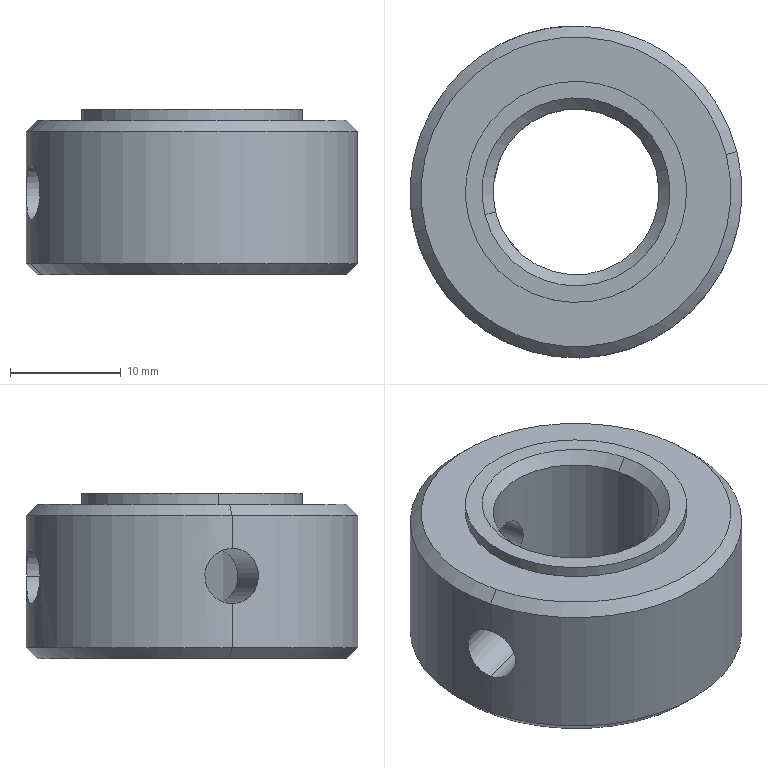Component | SolidWorks | KSD171005A-01-01-28-1 | 1 solid | 21 faces | box 30 x 30 x 15 mm | volume 7121 mm3 | cylinder 10 | cone 8 | plane 3 | commonest cylinder face diameters 5 x4 15 x2 20 x2 30 x2
build123d program:
from build123d import *

# Parameters (mm, degrees)
CHAMFER1_SIZE = 1
CHAMFER2_SIZE = 1
SKETCH2_W     = 2.5
SKETCH2_H     = 15
SKETCH4_W     = 2.5
SKETCH4_H     = 15


with BuildPart() as part:
    # Sketch1 → Revolve1 (revolve)
    with BuildSketch(Plane.XY, mode=Mode.PRIVATE) as revolve1_sk:
        Polygon((-7.5, 7.5), (7.5, 7.5), (7.5, 10), (6.5, 10), (6.5, 15), (-7.5, 15), align=None)
    revolve(revolve1_sk.sketch.rotate(Axis((0, 0, 0), (-1, 0, 0)), 90), axis=Axis((0, 0, 0), (-1, 0, 0)))

    # Chamfer1
    chamfer1_edges = [part.edges().sort_by_distance(p)[0] for p in [
        (6.5, 0, 15),
        (-7.5, 0, 15),
    ]]
    chamfer(chamfer1_edges, length=CHAMFER1_SIZE)

    # Chamfer2
    chamfer2_edges = [part.edges().sort_by_distance(p)[0] for p in [
        (-7.5, 0, 7.5),
        (7.5, 0, 7.5),
    ]]
    chamfer(chamfer2_edges, length=CHAMFER2_SIZE)

    # Sketch2 → M6 Tapped Hole1 (revolve, cut)
    with BuildSketch(Plane(origin=(0, 0, 0), x_dir=(0, 0, -1), z_dir=(1, 0, 0))):
        with Locations((1.25, 7.5)):
            Rectangle(SKETCH2_W, SKETCH2_H)
    revolve(axis=Axis((0, -6.35, 0), (0, 1, 0)), mode=Mode.SUBTRACT)

    # Sketch4 → M6 Tapped Hole2 (revolve, cut)
    with BuildSketch(Plane.YZ):
        with Locations((1.25, 7.5)):
            Rectangle(SKETCH4_W, SKETCH4_H)
    revolve(axis=Axis((0, 0, -6.35), (0, 0, 1)), mode=Mode.SUBTRACT)


solid = part.part

# Placed as in the assembly
solid = solid.moved(Location((-7.111, 15.73, 340.5), (90, -75.982, 90)))
STEP:
#1=COLOUR_RGB('',0.7922,0.8196,0.9333);
#2=FILL_AREA_STYLE_COLOUR('',#1);
#3=FILL_AREA_STYLE('',(#2));
#4=SURFACE_STYLE_FILL_AREA(#3);
#5=SURFACE_SIDE_STYLE('',(#4));
#6=SURFACE_STYLE_USAGE(.BOTH.,#5);
#7=PRESENTATION_STYLE_ASSIGNMENT((#6));
#8=CARTESIAN_POINT('',(-0.8529,0.4762,13.307));
#9=VERTEX_POINT('',#8);
#10=CARTESIAN_POINT('',(-0.8529,0.4762,13.504));
#11=VERTEX_POINT('',#10);
#12=CARTESIAN_POINT('',(-0.8529,0.4762,13.307));
#13=CARTESIAN_POINT('',(-0.8514,0.4699,13.307));
#14=CARTESIAN_POINT('',(-0.8497,0.4637,13.308));
#15=CARTESIAN_POINT('',(-0.8463,0.4516,13.31));
#16=CARTESIAN_POINT('',(-0.8444,0.4456,13.312));
#17=CARTESIAN_POINT('',(-0.8408,0.4342,13.317));
#18=CARTESIAN_POINT('',(-0.839,0.4288,13.32));
#19=CARTESIAN_POINT('',(-0.8354,0.4187,13.327));
#20=CARTESIAN_POINT('',(-0.8337,0.4139,13.331));
#21=CARTESIAN_POINT('',(-0.8288,0.4011,13.345));
#22=CARTESIAN_POINT('',(-0.826,0.3943,13.356));
#23=CARTESIAN_POINT('',(-0.8231,0.3874,13.374));
#24=CARTESIAN_POINT('',(-0.8224,0.3857,13.38));
#25=CARTESIAN_POINT('',(-0.8213,0.3833,13.393));
#26=CARTESIAN_POINT('',(-0.8211,0.3827,13.399));
#27=CARTESIAN_POINT('',(-0.8211,0.3827,13.412));
#28=CARTESIAN_POINT('',(-0.8213,0.3833,13.418));
#29=CARTESIAN_POINT('',(-0.8224,0.3857,13.431));
#30=CARTESIAN_POINT('',(-0.8231,0.3874,13.437));
#31=CARTESIAN_POINT('',(-0.825,0.392,13.449));
#32=CARTESIAN_POINT('',(-0.8262,0.3949,13.455));
#33=CARTESIAN_POINT('',(-0.8289,0.4015,13.466));
#34=CARTESIAN_POINT('',(-0.8304,0.4054,13.471));
#35=CARTESIAN_POINT('',(-0.8337,0.414,13.48));
#36=CARTESIAN_POINT('',(-0.8354,0.4187,13.484));
#37=CARTESIAN_POINT('',(-0.839,0.4288,13.491));
#38=CARTESIAN_POINT('',(-0.8408,0.4343,13.494));
#39=CARTESIAN_POINT('',(-0.8444,0.4456,13.499));
#40=CARTESIAN_POINT('',(-0.8462,0.4515,13.501));
#41=CARTESIAN_POINT('',(-0.8497,0.4637,13.503));
#42=CARTESIAN_POINT('',(-0.8514,0.47,13.504));
#43=CARTESIAN_POINT('',(-0.8529,0.4762,13.504));
#44=B_SPLINE_CURVE_WITH_KNOTS('',3,(#12,#13,#14,#15,#16,#17,#18,#19,#20,#21,#22,#23,#24,#25,#26,#27,#28,#29,#30,#31,#32,#33,#34,#35,#36,#37,#38,#39,#40,#41,#42,#43),.UNSPECIFIED.,.F.,.F.,(4,2,2,2,2,2,2,2,2,2,2,2,2,2,2,4),(0.,0.0004894,0.0009787,0.001468,0.001957,0.002936,0.003426,0.003915,0.004404,0.004894,0.005383,0.005872,0.006362,0.006851,0.00734,0.00783),.UNSPECIFIED.);
#45=EDGE_CURVE('',#9,#11,#44,.T.);
#46=ORIENTED_EDGE('',*,*,#45,.T.);
#47=CARTESIAN_POINT('',(-0.5665,0.5477,13.504));
#48=VERTEX_POINT('',#47);
#49=CARTESIAN_POINT('',(-0.28,0.6193,13.504));
#50=DIRECTION('',(0.9702,0.2423,0.));
#51=VECTOR('',#50,39.37);
#52=LINE('',#49,#51);
#53=EDGE_CURVE('',#11,#48,#52,.T.);
#54=ORIENTED_EDGE('',*,*,#53,.T.);
#55=CARTESIAN_POINT('',(-0.5665,0.5477,13.307));
#56=VERTEX_POINT('',#55);
#57=CARTESIAN_POINT('',(-0.5665,0.5477,13.504));
#58=CARTESIAN_POINT('',(-0.5649,0.5415,13.504));
#59=CARTESIAN_POINT('',(-0.5631,0.5352,13.503));
#60=CARTESIAN_POINT('',(-0.5592,0.523,13.501));
#61=CARTESIAN_POINT('',(-0.5571,0.5172,13.499));
#62=CARTESIAN_POINT('',(-0.5528,0.5061,13.494));
#63=CARTESIAN_POINT('',(-0.5505,0.5007,13.491));
#64=CARTESIAN_POINT('',(-0.5459,0.4909,13.484));
#65=CARTESIAN_POINT('',(-0.5437,0.4864,13.48));
#66=CARTESIAN_POINT('',(-0.5372,0.4739,13.466));
#67=CARTESIAN_POINT('',(-0.5333,0.4675,13.455));
#68=CARTESIAN_POINT('',(-0.5292,0.4608,13.437));
#69=CARTESIAN_POINT('',(-0.5281,0.4592,13.431));
#70=CARTESIAN_POINT('',(-0.5266,0.4569,13.419));
#71=CARTESIAN_POINT('',(-0.5262,0.4563,13.412));
#72=CARTESIAN_POINT('',(-0.5262,0.4563,13.399));
#73=CARTESIAN_POINT('',(-0.5266,0.4569,13.393));
#74=CARTESIAN_POINT('',(-0.5281,0.4592,13.38));
#75=CARTESIAN_POINT('',(-0.5292,0.4609,13.374));
#76=CARTESIAN_POINT('',(-0.5333,0.4675,13.356));
#77=CARTESIAN_POINT('',(-0.5372,0.474,13.345));
#78=CARTESIAN_POINT('',(-0.5437,0.4863,13.331));
#79=CARTESIAN_POINT('',(-0.546,0.4909,13.327));
#80=CARTESIAN_POINT('',(-0.5505,0.5008,13.32));
#81=CARTESIAN_POINT('',(-0.5527,0.506,13.317));
#82=CARTESIAN_POINT('',(-0.5571,0.5172,13.312));
#83=CARTESIAN_POINT('',(-0.5592,0.5231,13.31));
#84=CARTESIAN_POINT('',(-0.5631,0.5352,13.308));
#85=CARTESIAN_POINT('',(-0.5649,0.5414,13.307));
#86=CARTESIAN_POINT('',(-0.5665,0.5477,13.307));
#87=B_SPLINE_CURVE_WITH_KNOTS('',3,(#57,#58,#59,#60,#61,#62,#63,#64,#65,#66,#67,#68,#69,#70,#71,#72,#73,#74,#75,#76,#77,#78,#79,#80,#81,#82,#83,#84,#85,#86),.UNSPECIFIED.,.F.,.F.,(4,2,2,2,2,2,2,2,2,2,2,2,2,2,4),(0.007873,0.008365,0.008857,0.009349,0.009841,0.01082,0.01132,0.01181,0.0123,0.01279,0.01378,0.01427,0.01476,0.01525,0.01574),.UNSPECIFIED.);
#88=EDGE_CURVE('',#48,#56,#87,.T.);
#89=ORIENTED_EDGE('',*,*,#88,.T.);
#90=CARTESIAN_POINT('',(-0.28,0.6193,13.307));
#91=DIRECTION('',(0.9702,0.2423,0.));
#92=VECTOR('',#91,39.37);
#93=LINE('',#90,#92);
#94=EDGE_CURVE('',#9,#56,#93,.T.);
#95=ORIENTED_EDGE('',*,*,#94,.F.);
#96=EDGE_LOOP('',(#46,#54,#89,#95));
#97=FACE_OUTER_BOUND('',#96,.T.);
#98=CARTESIAN_POINT('',(-0.28,0.6193,13.406));
#99=DIRECTION('',(0.9702,0.2423,0.));
#100=DIRECTION('',(0.,0.,-1.));
#101=AXIS2_PLACEMENT_3D('',#98,#99,#100);
#102=CYLINDRICAL_SURFACE('',#101,0.09843);
#103=ADVANCED_FACE('',(#97),#102,.F.);
#104=CARTESIAN_POINT('',(-0.3255,1.208,13.406));
#105=VERTEX_POINT('',#104);
#106=CARTESIAN_POINT('',(-0.5165,1.16,13.406));
#107=VERTEX_POINT('',#106);
#108=CARTESIAN_POINT('',(-0.3255,1.208,13.406));
#109=CARTESIAN_POINT('',(-0.3255,1.208,13.399));
#110=CARTESIAN_POINT('',(-0.3262,1.208,13.393));
#111=CARTESIAN_POINT('',(-0.3287,1.208,13.38));
#112=CARTESIAN_POINT('',(-0.3306,1.208,13.374));
#113=CARTESIAN_POINT('',(-0.3356,1.207,13.362));
#114=CARTESIAN_POINT('',(-0.3387,1.207,13.356));
#115=CARTESIAN_POINT('',(-0.3458,1.206,13.345));
#116=CARTESIAN_POINT('',(-0.35,1.206,13.34));
#117=CARTESIAN_POINT('',(-0.3636,1.204,13.327));
#118=CARTESIAN_POINT('',(-0.3745,1.202,13.32));
#119=CARTESIAN_POINT('',(-0.392,1.199,13.312));
#120=CARTESIAN_POINT('',(-0.3981,1.198,13.31));
#121=CARTESIAN_POINT('',(-0.4105,1.195,13.308));
#122=CARTESIAN_POINT('',(-0.4168,1.194,13.307));
#123=CARTESIAN_POINT('',(-0.4292,1.191,13.307));
#124=CARTESIAN_POINT('',(-0.4356,1.189,13.308));
#125=CARTESIAN_POINT('',(-0.4477,1.186,13.31));
#126=CARTESIAN_POINT('',(-0.4536,1.184,13.312));
#127=CARTESIAN_POINT('',(-0.465,1.18,13.317));
#128=CARTESIAN_POINT('',(-0.4705,1.178,13.32));
#129=CARTESIAN_POINT('',(-0.4805,1.175,13.327));
#130=CARTESIAN_POINT('',(-0.4853,1.173,13.331));
#131=CARTESIAN_POINT('',(-0.4939,1.17,13.34));
#132=CARTESIAN_POINT('',(-0.4977,1.168,13.345));
#133=CARTESIAN_POINT('',(-0.5044,1.166,13.356));
#134=CARTESIAN_POINT('',(-0.5072,1.164,13.362));
#135=CARTESIAN_POINT('',(-0.5118,1.162,13.374));
#136=CARTESIAN_POINT('',(-0.5136,1.162,13.38));
#137=CARTESIAN_POINT('',(-0.5159,1.161,13.393));
#138=CARTESIAN_POINT('',(-0.5165,1.16,13.399));
#139=CARTESIAN_POINT('',(-0.5165,1.16,13.406));
#140=B_SPLINE_CURVE_WITH_KNOTS('',3,(#108,#109,#110,#111,#112,#113,#114,#115,#116,#117,#118,#119,#120,#121,#122,#123,#124,#125,#126,#127,#128,#129,#130,#131,#132,#133,#134,#135,#136,#137,#138,#139),.UNSPECIFIED.,.F.,.F.,(4,2,2,2,2,2,2,2,2,2,2,2,2,2,2,4),(0.,0.0004894,0.0009787,0.001468,0.001957,0.002936,0.003426,0.003915,0.004404,0.004894,0.005383,0.005872,0.006362,0.006851,0.00734,0.00783),.UNSPECIFIED.);
#141=EDGE_CURVE('',#105,#107,#140,.T.);
#142=ORIENTED_EDGE('',*,*,#141,.T.);
#143=CARTESIAN_POINT('',(-0.4429,0.8655,13.406));
#144=VERTEX_POINT('',#143);
#145=CARTESIAN_POINT('',(-0.3755,0.5954,13.406));
#146=DIRECTION('',(0.2423,-0.9702,0.));
#147=VECTOR('',#146,39.37);
#148=LINE('',#145,#147);
#149=EDGE_CURVE('',#107,#144,#148,.T.);
#150=ORIENTED_EDGE('',*,*,#149,.T.);
#151=CARTESIAN_POINT('',(-0.2519,0.9132,13.406));
#152=VERTEX_POINT('',#151);
#153=CARTESIAN_POINT('',(-0.4429,0.8655,13.406));
#154=CARTESIAN_POINT('',(-0.4429,0.8655,13.399));
#155=CARTESIAN_POINT('',(-0.4423,0.8659,13.393));
#156=CARTESIAN_POINT('',(-0.4401,0.8674,13.38));
#157=CARTESIAN_POINT('',(-0.4384,0.8685,13.374));
#158=CARTESIAN_POINT('',(-0.434,0.8712,13.362));
#159=CARTESIAN_POINT('',(-0.4312,0.8729,13.356));
#160=CARTESIAN_POINT('',(-0.4248,0.8766,13.345));
#161=CARTESIAN_POINT('',(-0.4212,0.8787,13.34));
#162=CARTESIAN_POINT('',(-0.4087,0.8852,13.327));
#163=CARTESIAN_POINT('',(-0.3988,0.8898,13.32));
#164=CARTESIAN_POINT('',(-0.382,0.8964,13.312));
#165=CARTESIAN_POINT('',(-0.3762,0.8985,13.31));
#166=CARTESIAN_POINT('',(-0.3641,0.9024,13.308));
#167=CARTESIAN_POINT('',(-0.3578,0.9042,13.307));
#168=CARTESIAN_POINT('',(-0.3452,0.9073,13.307));
#169=CARTESIAN_POINT('',(-0.3389,0.9087,13.308));
#170=CARTESIAN_POINT('',(-0.3264,0.911,13.31));
#171=CARTESIAN_POINT('',(-0.3201,0.9119,13.312));
#172=CARTESIAN_POINT('',(-0.3023,0.914,13.32));
#173=CARTESIAN_POINT('',(-0.2912,0.9145,13.327));
#174=CARTESIAN_POINT('',(-0.2773,0.9146,13.34));
#175=CARTESIAN_POINT('',(-0.273,0.9145,13.345));
#176=CARTESIAN_POINT('',(-0.2656,0.9142,13.356));
#177=CARTESIAN_POINT('',(-0.2625,0.914,13.362));
#178=CARTESIAN_POINT('',(-0.2573,0.9137,13.374));
#179=CARTESIAN_POINT('',(-0.2553,0.9135,13.38));
#180=CARTESIAN_POINT('',(-0.2526,0.9133,13.393));
#181=CARTESIAN_POINT('',(-0.2519,0.9132,13.399));
#182=CARTESIAN_POINT('',(-0.2519,0.9132,13.406));
#183=B_SPLINE_CURVE_WITH_KNOTS('',3,(#153,#154,#155,#156,#157,#158,#159,#160,#161,#162,#163,#164,#165,#166,#167,#168,#169,#170,#171,#172,#173,#174,#175,#176,#177,#178,#179,#180,#181,#182),.UNSPECIFIED.,.F.,.F.,(4,2,2,2,2,2,2,2,2,2,2,2,2,2,4),(0.007873,0.008365,0.008857,0.009348,0.00984,0.01082,0.01132,0.01181,0.0123,0.01279,0.01378,0.01427,0.01476,0.01525,0.01574),.UNSPECIFIED.);
#184=EDGE_CURVE('',#144,#152,#183,.T.);
#185=ORIENTED_EDGE('',*,*,#184,.T.);
#186=CARTESIAN_POINT('',(-0.1845,0.6431,13.406));
#187=DIRECTION('',(0.2423,-0.9702,0.));
#188=VECTOR('',#187,39.37);
#189=LINE('',#186,#188);
#190=EDGE_CURVE('',#105,#152,#189,.T.);
#191=ORIENTED_EDGE('',*,*,#190,.F.);
#192=EDGE_LOOP('',(#142,#150,#185,#191));
#193=FACE_OUTER_BOUND('',#192,.T.);
#194=CARTESIAN_POINT('',(-0.28,0.6193,13.406));
#195=DIRECTION('',(0.2423,-0.9702,0.));
#196=DIRECTION('',(0.9702,0.2423,0.));
#197=AXIS2_PLACEMENT_3D('',#194,#195,#196);
#198=CYLINDRICAL_SURFACE('',#197,0.09843);
#199=ADVANCED_FACE('',(#193),#198,.F.);
#200=CARTESIAN_POINT('',(0.006506,0.6908,13.15));
#201=VERTEX_POINT('',#200);
#202=CARTESIAN_POINT('',(-0.5665,0.5477,13.15));
#203=VERTEX_POINT('',#202);
#204=CARTESIAN_POINT('',(-0.28,0.6193,13.15));
#205=DIRECTION('',(0.,0.,-1.));
#206=DIRECTION('',(-0.9702,-0.2423,0.));
#207=AXIS2_PLACEMENT_3D('',#204,#205,#206);
#208=CIRCLE('',#207,0.2953);
#209=EDGE_CURVE('',#201,#203,#208,.T.);
#210=ORIENTED_EDGE('',*,*,#209,.F.);
#211=CARTESIAN_POINT('',(0.0447,0.7004,13.11));
#212=VERTEX_POINT('',#211);
#213=CARTESIAN_POINT('',(0.0447,0.7004,13.11));
#214=DIRECTION('',(0.686,0.1713,-0.7071));
#215=VECTOR('',#214,39.37);
#216=LINE('',#213,#215);
#217=EDGE_CURVE('',#201,#212,#216,.T.);
#218=ORIENTED_EDGE('',*,*,#217,.T.);
#219=CARTESIAN_POINT('',(-0.6047,0.5382,13.11));
#220=VERTEX_POINT('',#219);
#221=CARTESIAN_POINT('',(-0.28,0.6193,13.11));
#222=DIRECTION('',(0.,0.,1.));
#223=DIRECTION('',(-0.9702,-0.2423,0.));
#224=AXIS2_PLACEMENT_3D('',#221,#222,#223);
#225=CIRCLE('',#224,0.3346);
#226=EDGE_CURVE('',#220,#212,#225,.T.);
#227=ORIENTED_EDGE('',*,*,#226,.F.);
#228=CARTESIAN_POINT('',(-0.6047,0.5382,13.11));
#229=DIRECTION('',(-0.686,-0.1713,-0.7071));
#230=VECTOR('',#229,39.37);
#231=LINE('',#228,#230);
#232=EDGE_CURVE('',#203,#220,#231,.T.);
#233=ORIENTED_EDGE('',*,*,#232,.F.);
#234=EDGE_LOOP('',(#210,#218,#227,#233));
#235=FACE_OUTER_BOUND('',#234,.T.);
#236=CARTESIAN_POINT('',(-0.28,0.6193,13.11));
#237=DIRECTION('',(0.,0.,-1.));
#238=DIRECTION('',(-0.9702,-0.2423,0.));
#239=AXIS2_PLACEMENT_3D('',#236,#237,#238);
#240=CONICAL_SURFACE('',#239,0.3346,0.7854);
#241=ADVANCED_FACE('',(#235),#240,.F.);
#242=CARTESIAN_POINT('',(-0.5665,0.5477,13.661));
#243=VERTEX_POINT('',#242);
#244=CARTESIAN_POINT('',(0.006506,0.6908,13.661));
#245=VERTEX_POINT('',#244);
#246=CARTESIAN_POINT('',(-0.28,0.6193,13.661));
#247=DIRECTION('',(0.,0.,1.));
#248=DIRECTION('',(0.9702,0.2423,0.));
#249=AXIS2_PLACEMENT_3D('',#246,#247,#248);
#250=CIRCLE('',#249,0.2953);
#251=EDGE_CURVE('',#243,#245,#250,.T.);
#252=ORIENTED_EDGE('',*,*,#251,.F.);
#253=CARTESIAN_POINT('',(-0.6047,0.5382,13.701));
#254=VERTEX_POINT('',#253);
#255=CARTESIAN_POINT('',(-0.5665,0.5477,13.661));
#256=DIRECTION('',(-0.686,-0.1713,0.7071));
#257=VECTOR('',#256,39.37);
#258=LINE('',#255,#257);
#259=EDGE_CURVE('',#243,#254,#258,.T.);
#260=ORIENTED_EDGE('',*,*,#259,.T.);
#261=CARTESIAN_POINT('',(0.0447,0.7004,13.701));
#262=VERTEX_POINT('',#261);
#263=CARTESIAN_POINT('',(-0.28,0.6193,13.701));
#264=DIRECTION('',(0.,0.,-1.));
#265=DIRECTION('',(0.9702,0.2423,0.));
#266=AXIS2_PLACEMENT_3D('',#263,#264,#265);
#267=CIRCLE('',#266,0.3346);
#268=EDGE_CURVE('',#262,#254,#267,.T.);
#269=ORIENTED_EDGE('',*,*,#268,.F.);
#270=CARTESIAN_POINT('',(0.006506,0.6908,13.661));
#271=DIRECTION('',(0.686,0.1713,0.7071));
#272=VECTOR('',#271,39.37);
#273=LINE('',#270,#272);
#274=EDGE_CURVE('',#245,#262,#273,.T.);
#275=ORIENTED_EDGE('',*,*,#274,.F.);
#276=EDGE_LOOP('',(#252,#260,#269,#275));
#277=FACE_OUTER_BOUND('',#276,.T.);
#278=CARTESIAN_POINT('',(-0.28,0.6193,13.661));
#279=DIRECTION('',(0.,0.,1.));
#280=DIRECTION('',(0.9702,0.2423,0.));
#281=AXIS2_PLACEMENT_3D('',#278,#279,#280);
#282=CONICAL_SURFACE('',#281,0.2953,0.7854);
#283=ADVANCED_FACE('',(#277),#282,.F.);
#284=CARTESIAN_POINT('',(-0.8147,0.4858,13.11));
#285=VERTEX_POINT('',#284);
#286=CARTESIAN_POINT('',(0.2548,0.7528,13.11));
#287=VERTEX_POINT('',#286);
#288=CARTESIAN_POINT('',(-0.28,0.6193,13.11));
#289=DIRECTION('',(0.,0.,-1.));
#290=DIRECTION('',(-0.9702,-0.2423,0.));
#291=AXIS2_PLACEMENT_3D('',#288,#289,#290);
#292=CIRCLE('',#291,0.5512);
#293=EDGE_CURVE('',#285,#287,#292,.T.);
#294=ORIENTED_EDGE('',*,*,#293,.F.);
#295=CARTESIAN_POINT('',(-0.8529,0.4762,13.15));
#296=VERTEX_POINT('',#295);
#297=CARTESIAN_POINT('',(-0.8529,0.4762,13.15));
#298=DIRECTION('',(-0.686,-0.1713,0.7071));
#299=VECTOR('',#298,39.37);
#300=LINE('',#297,#299);
#301=EDGE_CURVE('',#285,#296,#300,.T.);
#302=ORIENTED_EDGE('',*,*,#301,.T.);
#303=CARTESIAN_POINT('',(0.293,0.7623,13.15));
#304=VERTEX_POINT('',#303);
#305=CARTESIAN_POINT('',(-0.28,0.6193,13.15));
#306=DIRECTION('',(0.,0.,1.));
#307=DIRECTION('',(-0.9702,-0.2423,0.));
#308=AXIS2_PLACEMENT_3D('',#305,#306,#307);
#309=CIRCLE('',#308,0.5906);
#310=EDGE_CURVE('',#304,#296,#309,.T.);
#311=ORIENTED_EDGE('',*,*,#310,.F.);
#312=CARTESIAN_POINT('',(0.293,0.7623,13.15));
#313=DIRECTION('',(0.686,0.1713,0.7071));
#314=VECTOR('',#313,39.37);
#315=LINE('',#312,#314);
#316=EDGE_CURVE('',#287,#304,#315,.T.);
#317=ORIENTED_EDGE('',*,*,#316,.F.);
#318=EDGE_LOOP('',(#294,#302,#311,#317));
#319=FACE_OUTER_BOUND('',#318,.T.);
#320=CARTESIAN_POINT('',(-0.28,0.6193,13.15));
#321=DIRECTION('',(0.,0.,1.));
#322=DIRECTION('',(0.9702,0.2423,0.));
#323=AXIS2_PLACEMENT_3D('',#320,#321,#322);
#324=CONICAL_SURFACE('',#323,0.5906,0.7854);
#325=ADVANCED_FACE('',(#319),#324,.T.);
#326=CARTESIAN_POINT('',(0.2548,0.7528,13.661));
#327=VERTEX_POINT('',#326);
#328=CARTESIAN_POINT('',(-0.8147,0.4858,13.661));
#329=VERTEX_POINT('',#328);
#330=CARTESIAN_POINT('',(-0.28,0.6193,13.661));
#331=DIRECTION('',(0.,0.,1.));
#332=DIRECTION('',(0.9702,0.2423,0.));
#333=AXIS2_PLACEMENT_3D('',#330,#331,#332);
#334=CIRCLE('',#333,0.5512);
#335=EDGE_CURVE('',#327,#329,#334,.T.);
#336=ORIENTED_EDGE('',*,*,#335,.F.);
#337=CARTESIAN_POINT('',(0.293,0.7623,13.622));
#338=VERTEX_POINT('',#337);
#339=CARTESIAN_POINT('',(0.2548,0.7528,13.661));
#340=DIRECTION('',(0.686,0.1713,-0.7071));
#341=VECTOR('',#340,39.37);
#342=LINE('',#339,#341);
#343=EDGE_CURVE('',#327,#338,#342,.T.);
#344=ORIENTED_EDGE('',*,*,#343,.T.);
#345=CARTESIAN_POINT('',(-0.8529,0.4762,13.622));
#346=VERTEX_POINT('',#345);
#347=CARTESIAN_POINT('',(-0.28,0.6193,13.622));
#348=DIRECTION('',(0.,0.,-1.));
#349=DIRECTION('',(0.9702,0.2423,0.));
#350=AXIS2_PLACEMENT_3D('',#347,#348,#349);
#351=CIRCLE('',#350,0.5906);
#352=EDGE_CURVE('',#346,#338,#351,.T.);
#353=ORIENTED_EDGE('',*,*,#352,.F.);
#354=CARTESIAN_POINT('',(-0.8147,0.4858,13.661));
#355=DIRECTION('',(-0.686,-0.1713,-0.7071));
#356=VECTOR('',#355,39.37);
#357=LINE('',#354,#356);
#358=EDGE_CURVE('',#329,#346,#357,.T.);
#359=ORIENTED_EDGE('',*,*,#358,.F.);
#360=EDGE_LOOP('',(#336,#344,#353,#359));
#361=FACE_OUTER_BOUND('',#360,.T.);
#362=CARTESIAN_POINT('',(-0.28,0.6193,13.661));
#363=DIRECTION('',(0.,0.,-1.));
#364=DIRECTION('',(-0.9702,-0.2423,0.));
#365=AXIS2_PLACEMENT_3D('',#362,#363,#364);
#366=CONICAL_SURFACE('',#365,0.5512,0.7854);
#367=ADVANCED_FACE('',(#361),#366,.T.);
#368=ORIENTED_EDGE('',*,*,#209,.T.);
#369=CARTESIAN_POINT('',(-0.5665,0.5477,13.406));
#370=DIRECTION('',(0.,0.,1.));
#371=VECTOR('',#370,39.37);
#372=LINE('',#369,#371);
#373=EDGE_CURVE('',#203,#56,#372,.T.);
#374=ORIENTED_EDGE('',*,*,#373,.T.);
#375=ORIENTED_EDGE('',*,*,#88,.F.);
#376=CARTESIAN_POINT('',(-0.5665,0.5477,13.406));
#377=DIRECTION('',(0.,0.,1.));
#378=VECTOR('',#377,39.37);
#379=LINE('',#376,#378);
#380=EDGE_CURVE('',#48,#243,#379,.T.);
#381=ORIENTED_EDGE('',*,*,#380,.T.);
#382=ORIENTED_EDGE('',*,*,#251,.T.);
#383=CARTESIAN_POINT('',(0.006506,0.6908,13.406));
#384=DIRECTION('',(0.,0.,1.));
#385=VECTOR('',#384,39.37);
#386=LINE('',#383,#385);
#387=EDGE_CURVE('',#201,#245,#386,.T.);
#388=ORIENTED_EDGE('',*,*,#387,.F.);
#389=EDGE_LOOP('',(#368,#374,#375,#381,#382,#388));
#390=FACE_OUTER_BOUND('',#389,.T.);
#391=CARTESIAN_POINT('',(-0.28,0.6193,13.406));
#392=DIRECTION('',(0.,0.,1.));
#393=DIRECTION('',(0.9702,0.2423,0.));
#394=AXIS2_PLACEMENT_3D('',#391,#392,#393);
#395=CYLINDRICAL_SURFACE('',#394,0.2953);
#396=ADVANCED_FACE('',(#390),#395,.F.);
#397=CARTESIAN_POINT('',(0.102,0.7147,13.661));
#398=VERTEX_POINT('',#397);
#399=CARTESIAN_POINT('',(-0.6619,0.5239,13.661));
#400=VERTEX_POINT('',#399);
#401=CARTESIAN_POINT('',(-0.28,0.6193,13.661));
#402=DIRECTION('',(0.,0.,1.));
#403=DIRECTION('',(0.9702,0.2423,0.));
#404=AXIS2_PLACEMENT_3D('',#401,#402,#403);
#405=CIRCLE('',#404,0.3937);
#406=EDGE_CURVE('',#398,#400,#405,.T.);
#407=ORIENTED_EDGE('',*,*,#406,.T.);
#408=CARTESIAN_POINT('',(-0.6619,0.5239,13.701));
#409=VERTEX_POINT('',#408);
#410=CARTESIAN_POINT('',(-0.6619,0.5239,13.406));
#411=DIRECTION('',(0.,0.,1.));
#412=VECTOR('',#411,39.37);
#413=LINE('',#410,#412);
#414=EDGE_CURVE('',#400,#409,#413,.T.);
#415=ORIENTED_EDGE('',*,*,#414,.T.);
#416=CARTESIAN_POINT('',(0.102,0.7147,13.701));
#417=VERTEX_POINT('',#416);
#418=CARTESIAN_POINT('',(-0.28,0.6193,13.701));
#419=DIRECTION('',(0.,0.,1.));
#420=DIRECTION('',(0.9702,0.2423,0.));
#421=AXIS2_PLACEMENT_3D('',#418,#419,#420);
#422=CIRCLE('',#421,0.3937);
#423=EDGE_CURVE('',#417,#409,#422,.T.);
#424=ORIENTED_EDGE('',*,*,#423,.F.);
#425=CARTESIAN_POINT('',(0.102,0.7147,13.406));
#426=DIRECTION('',(0.,0.,1.));
#427=VECTOR('',#426,39.37);
#428=LINE('',#425,#427);
#429=EDGE_CURVE('',#398,#417,#428,.T.);
#430=ORIENTED_EDGE('',*,*,#429,.F.);
#431=EDGE_LOOP('',(#407,#415,#424,#430));
#432=FACE_OUTER_BOUND('',#431,.T.);
#433=CARTESIAN_POINT('',(-0.28,0.6193,13.406));
#434=DIRECTION('',(0.,0.,1.));
#435=DIRECTION('',(0.9702,0.2423,0.));
#436=AXIS2_PLACEMENT_3D('',#433,#434,#435);
#437=CYLINDRICAL_SURFACE('',#436,0.3937);
#438=ADVANCED_FACE('',(#432),#437,.T.);
#439=ORIENTED_EDGE('',*,*,#141,.F.);
#440=CARTESIAN_POINT('',(-0.5165,1.16,13.406));
#441=CARTESIAN_POINT('',(-0.5165,1.16,13.418));
#442=CARTESIAN_POINT('',(-0.5141,1.161,13.431));
#443=CARTESIAN_POINT('',(-0.5073,1.164,13.449));
#444=CARTESIAN_POINT('',(-0.5044,1.166,13.455));
#445=CARTESIAN_POINT('',(-0.4977,1.168,13.466));
#446=CARTESIAN_POINT('',(-0.4939,1.17,13.471));
#447=CARTESIAN_POINT('',(-0.4853,1.173,13.48));
#448=CARTESIAN_POINT('',(-0.4806,1.175,13.484));
#449=CARTESIAN_POINT('',(-0.4705,1.178,13.491));
#450=CARTESIAN_POINT('',(-0.4651,1.18,13.494));
#451=CARTESIAN_POINT('',(-0.4537,1.184,13.499));
#452=CARTESIAN_POINT('',(-0.4477,1.186,13.501));
#453=CARTESIAN_POINT('',(-0.4356,1.189,13.503));
#454=CARTESIAN_POINT('',(-0.4294,1.191,13.504));
#455=CARTESIAN_POINT('',(-0.4168,1.194,13.504));
#456=CARTESIAN_POINT('',(-0.4106,1.195,13.503));
#457=CARTESIAN_POINT('',(-0.3982,1.198,13.501));
#458=CARTESIAN_POINT('',(-0.3921,1.199,13.499));
#459=CARTESIAN_POINT('',(-0.3803,1.201,13.494));
#460=CARTESIAN_POINT('',(-0.3747,1.202,13.491));
#461=CARTESIAN_POINT('',(-0.3641,1.204,13.484));
#462=CARTESIAN_POINT('',(-0.3591,1.205,13.48));
#463=CARTESIAN_POINT('',(-0.3455,1.206,13.466));
#464=CARTESIAN_POINT('',(-0.3381,1.207,13.455));
#465=CARTESIAN_POINT('',(-0.3307,1.208,13.437));
#466=CARTESIAN_POINT('',(-0.3288,1.208,13.431));
#467=CARTESIAN_POINT('',(-0.3262,1.208,13.418));
#468=CARTESIAN_POINT('',(-0.3255,1.208,13.412));
#469=CARTESIAN_POINT('',(-0.3255,1.208,13.406));
#470=B_SPLINE_CURVE_WITH_KNOTS('',3,(#440,#441,#442,#443,#444,#445,#446,#447,#448,#449,#450,#451,#452,#453,#454,#455,#456,#457,#458,#459,#460,#461,#462,#463,#464,#465,#466,#467,#468,#469),.UNSPECIFIED.,.F.,.F.,(4,2,2,2,2,2,2,2,2,2,2,2,2,2,4),(0.00783,0.008808,0.009298,0.009787,0.01028,0.01077,0.01125,0.01174,0.01223,0.01272,0.01321,0.0137,0.01468,0.01517,0.01566),.UNSPECIFIED.);
#471=EDGE_CURVE('',#107,#105,#470,.T.);
#472=ORIENTED_EDGE('',*,*,#471,.F.);
#473=EDGE_LOOP('',(#439,#472));
#474=FACE_BOUND('',#473,.T.);
#475=ORIENTED_EDGE('',*,*,#310,.T.);
#476=CARTESIAN_POINT('',(-0.8529,0.4762,13.406));
#477=DIRECTION('',(0.,0.,1.));
#478=VECTOR('',#477,39.37);
#479=LINE('',#476,#478);
#480=EDGE_CURVE('',#296,#9,#479,.T.);
#481=ORIENTED_EDGE('',*,*,#480,.T.);
#482=CARTESIAN_POINT('',(-0.8529,0.4762,13.504));
#483=CARTESIAN_POINT('',(-0.856,0.4887,13.504));
#484=CARTESIAN_POINT('',(-0.8588,0.5014,13.501));
#485=CARTESIAN_POINT('',(-0.862,0.5189,13.494));
#486=CARTESIAN_POINT('',(-0.8629,0.5246,13.491));
#487=CARTESIAN_POINT('',(-0.8645,0.5352,13.484));
#488=CARTESIAN_POINT('',(-0.8652,0.5402,13.48));
#489=CARTESIAN_POINT('',(-0.8664,0.5492,13.471));
#490=CARTESIAN_POINT('',(-0.8668,0.5534,13.466));
#491=CARTESIAN_POINT('',(-0.8676,0.5606,13.455));
#492=CARTESIAN_POINT('',(-0.8679,0.5636,13.449));
#493=CARTESIAN_POINT('',(-0.8684,0.5686,13.437));
#494=CARTESIAN_POINT('',(-0.8685,0.5705,13.431));
#495=CARTESIAN_POINT('',(-0.8687,0.5731,13.419));
#496=CARTESIAN_POINT('',(-0.8688,0.5737,13.412));
#497=CARTESIAN_POINT('',(-0.8688,0.5737,13.399));
#498=CARTESIAN_POINT('',(-0.8687,0.5731,13.393));
#499=CARTESIAN_POINT('',(-0.8685,0.5705,13.38));
#500=CARTESIAN_POINT('',(-0.8684,0.5686,13.374));
#501=CARTESIAN_POINT('',(-0.8679,0.5637,13.362));
#502=CARTESIAN_POINT('',(-0.8676,0.5606,13.356));
#503=CARTESIAN_POINT('',(-0.8669,0.5535,13.346));
#504=CARTESIAN_POINT('',(-0.8664,0.5493,13.34));
#505=CARTESIAN_POINT('',(-0.8647,0.5357,13.327));
#506=CARTESIAN_POINT('',(-0.863,0.5249,13.32));
#507=CARTESIAN_POINT('',(-0.8599,0.5074,13.312));
#508=CARTESIAN_POINT('',(-0.8586,0.5012,13.31));
#509=CARTESIAN_POINT('',(-0.856,0.4888,13.308));
#510=CARTESIAN_POINT('',(-0.8545,0.4825,13.307));
#511=CARTESIAN_POINT('',(-0.8529,0.4762,13.307));
#512=B_SPLINE_CURVE_WITH_KNOTS('',3,(#482,#483,#484,#485,#486,#487,#488,#489,#490,#491,#492,#493,#494,#495,#496,#497,#498,#499,#500,#501,#502,#503,#504,#505,#506,#507,#508,#509,#510,#511),.UNSPECIFIED.,.F.,.F.,(4,2,2,2,2,2,2,2,2,2,2,2,2,2,4),(0.00783,0.008808,0.009298,0.009787,0.01028,0.01077,0.01125,0.01174,0.01223,0.01272,0.01321,0.0137,0.01468,0.01517,0.01566),.UNSPECIFIED.);
#513=EDGE_CURVE('',#11,#9,#512,.T.);
#514=ORIENTED_EDGE('',*,*,#513,.F.);
#515=CARTESIAN_POINT('',(-0.8529,0.4762,13.406));
#516=DIRECTION('',(0.,0.,1.));
#517=VECTOR('',#516,39.37);
#518=LINE('',#515,#517);
#519=EDGE_CURVE('',#11,#346,#518,.T.);
#520=ORIENTED_EDGE('',*,*,#519,.T.);
#521=ORIENTED_EDGE('',*,*,#352,.T.);
#522=CARTESIAN_POINT('',(0.293,0.7623,13.406));
#523=DIRECTION('',(0.,0.,1.));
#524=VECTOR('',#523,39.37);
#525=LINE('',#522,#524);
#526=EDGE_CURVE('',#304,#338,#525,.T.);
#527=ORIENTED_EDGE('',*,*,#526,.F.);
#528=EDGE_LOOP('',(#475,#481,#514,#520,#521,#527));
#529=FACE_OUTER_BOUND('',#528,.T.);
#530=CARTESIAN_POINT('',(-0.28,0.6193,13.406));
#531=DIRECTION('',(0.,0.,1.));
#532=DIRECTION('',(0.9702,0.2423,0.));
#533=AXIS2_PLACEMENT_3D('',#530,#531,#532);
#534=CYLINDRICAL_SURFACE('',#533,0.5906);
#535=ADVANCED_FACE('',(#474,#529),#534,.T.);
#536=ORIENTED_EDGE('',*,*,#226,.T.);
#537=CARTESIAN_POINT('',(-0.28,0.6193,13.11));
#538=DIRECTION('',(0.,0.,1.));
#539=DIRECTION('',(-0.9702,-0.2423,0.));
#540=AXIS2_PLACEMENT_3D('',#537,#538,#539);
#541=CIRCLE('',#540,0.3346);
#542=EDGE_CURVE('',#212,#220,#541,.T.);
#543=ORIENTED_EDGE('',*,*,#542,.T.);
#544=EDGE_LOOP('',(#536,#543));
#545=FACE_BOUND('',#544,.T.);
#546=CARTESIAN_POINT('',(-0.28,0.6193,13.11));
#547=DIRECTION('',(0.,0.,-1.));
#548=DIRECTION('',(-0.9702,-0.2423,0.));
#549=AXIS2_PLACEMENT_3D('',#546,#547,#548);
#550=CIRCLE('',#549,0.5512);
#551=EDGE_CURVE('',#287,#285,#550,.T.);
#552=ORIENTED_EDGE('',*,*,#551,.T.);
#553=ORIENTED_EDGE('',*,*,#293,.T.);
#554=EDGE_LOOP('',(#552,#553));
#555=FACE_OUTER_BOUND('',#554,.T.);
#556=CARTESIAN_POINT('',(-0.3515,0.9058,13.11));
#557=DIRECTION('',(0.,0.,-1.));
#558=DIRECTION('',(-0.9702,-0.2423,-0.));
#559=AXIS2_PLACEMENT_3D('',#556,#557,#558);
#560=PLANE('',#559);
#561=ADVANCED_FACE('',(#545,#555),#560,.T.);
#562=ORIENTED_EDGE('',*,*,#480,.F.);
#563=CARTESIAN_POINT('',(-0.28,0.6193,13.15));
#564=DIRECTION('',(0.,0.,1.));
#565=DIRECTION('',(-0.9702,-0.2423,0.));
#566=AXIS2_PLACEMENT_3D('',#563,#564,#565);
#567=CIRCLE('',#566,0.5906);
#568=EDGE_CURVE('',#296,#304,#567,.T.);
#569=ORIENTED_EDGE('',*,*,#568,.T.);
#570=ORIENTED_EDGE('',*,*,#526,.T.);
#571=CARTESIAN_POINT('',(-0.28,0.6193,13.622));
#572=DIRECTION('',(0.,0.,-1.));
#573=DIRECTION('',(0.9702,0.2423,0.));
#574=AXIS2_PLACEMENT_3D('',#571,#572,#573);
#575=CIRCLE('',#574,0.5906);
#576=EDGE_CURVE('',#338,#346,#575,.T.);
#577=ORIENTED_EDGE('',*,*,#576,.T.);
#578=ORIENTED_EDGE('',*,*,#519,.F.);
#579=ORIENTED_EDGE('',*,*,#45,.F.);
#580=EDGE_LOOP('',(#562,#569,#570,#577,#578,#579));
#581=FACE_OUTER_BOUND('',#580,.T.);
#582=CARTESIAN_POINT('',(-0.28,0.6193,13.406));
#583=DIRECTION('',(0.,0.,1.));
#584=DIRECTION('',(0.9702,0.2423,0.));
#585=AXIS2_PLACEMENT_3D('',#582,#583,#584);
#586=CYLINDRICAL_SURFACE('',#585,0.5906);
#587=ADVANCED_FACE('',(#581),#586,.T.);
#588=CARTESIAN_POINT('',(-0.28,0.6193,13.661));
#589=DIRECTION('',(0.,0.,1.));
#590=DIRECTION('',(0.9702,0.2423,0.));
#591=AXIS2_PLACEMENT_3D('',#588,#589,#590);
#592=CIRCLE('',#591,0.5512);
#593=EDGE_CURVE('',#329,#327,#592,.T.);
#594=ORIENTED_EDGE('',*,*,#593,.T.);
#595=ORIENTED_EDGE('',*,*,#335,.T.);
#596=EDGE_LOOP('',(#594,#595));
#597=FACE_OUTER_BOUND('',#596,.T.);
#598=ORIENTED_EDGE('',*,*,#406,.F.);
#599=CARTESIAN_POINT('',(-0.28,0.6193,13.661));
#600=DIRECTION('',(0.,0.,1.));
#601=DIRECTION('',(0.9702,0.2423,0.));
#602=AXIS2_PLACEMENT_3D('',#599,#600,#601);
#603=CIRCLE('',#602,0.3937);
#604=EDGE_CURVE('',#400,#398,#603,.T.);
#605=ORIENTED_EDGE('',*,*,#604,.F.);
#606=EDGE_LOOP('',(#598,#605));
#607=FACE_BOUND('',#606,.T.);
#608=CARTESIAN_POINT('',(-0.423,1.192,13.661));
#609=DIRECTION('',(-0.,-0.,1.));
#610=DIRECTION('',(0.9702,0.2423,0.));
#611=AXIS2_PLACEMENT_3D('',#608,#609,#610);
#612=PLANE('',#611);
#613=ADVANCED_FACE('',(#597,#607),#612,.T.);
#614=ORIENTED_EDGE('',*,*,#414,.F.);
#615=ORIENTED_EDGE('',*,*,#604,.T.);
#616=ORIENTED_EDGE('',*,*,#429,.T.);
#617=CARTESIAN_POINT('',(-0.28,0.6193,13.701));
#618=DIRECTION('',(0.,0.,1.));
#619=DIRECTION('',(0.9702,0.2423,0.));
#620=AXIS2_PLACEMENT_3D('',#617,#618,#619);
#621=CIRCLE('',#620,0.3937);
#622=EDGE_CURVE('',#409,#417,#621,.T.);
#623=ORIENTED_EDGE('',*,*,#622,.F.);
#624=EDGE_LOOP('',(#614,#615,#616,#623));
#625=FACE_OUTER_BOUND('',#624,.T.);
#626=CARTESIAN_POINT('',(-0.28,0.6193,13.406));
#627=DIRECTION('',(0.,0.,1.));
#628=DIRECTION('',(0.9702,0.2423,0.));
#629=AXIS2_PLACEMENT_3D('',#626,#627,#628);
#630=CYLINDRICAL_SURFACE('',#629,0.3937);
#631=ADVANCED_FACE('',(#625),#630,.T.);
#632=ORIENTED_EDGE('',*,*,#268,.T.);
#633=CARTESIAN_POINT('',(-0.28,0.6193,13.701));
#634=DIRECTION('',(0.,0.,-1.));
#635=DIRECTION('',(0.9702,0.2423,0.));
#636=AXIS2_PLACEMENT_3D('',#633,#634,#635);
#637=CIRCLE('',#636,0.3346);
#638=EDGE_CURVE('',#254,#262,#637,.T.);
#639=ORIENTED_EDGE('',*,*,#638,.T.);
#640=EDGE_LOOP('',(#632,#639));
#641=FACE_BOUND('',#640,.T.);
#642=ORIENTED_EDGE('',*,*,#423,.T.);
#643=ORIENTED_EDGE('',*,*,#622,.T.);
#644=EDGE_LOOP('',(#642,#643));
#645=FACE_OUTER_BOUND('',#644,.T.);
#646=CARTESIAN_POINT('',(-0.3515,0.9058,13.701));
#647=DIRECTION('',(-0.,-0.,1.));
#648=DIRECTION('',(0.9702,0.2423,0.));
#649=AXIS2_PLACEMENT_3D('',#646,#647,#648);
#650=PLANE('',#649);
#651=ADVANCED_FACE('',(#641,#645),#650,.T.);
#652=ORIENTED_EDGE('',*,*,#373,.F.);
#653=CARTESIAN_POINT('',(-0.28,0.6193,13.15));
#654=DIRECTION('',(0.,0.,-1.));
#655=DIRECTION('',(-0.9702,-0.2423,0.));
#656=AXIS2_PLACEMENT_3D('',#653,#654,#655);
#657=CIRCLE('',#656,0.2953);
#658=EDGE_CURVE('',#203,#201,#657,.T.);
#659=ORIENTED_EDGE('',*,*,#658,.T.);
#660=ORIENTED_EDGE('',*,*,#387,.T.);
#661=CARTESIAN_POINT('',(-0.28,0.6193,13.661));
#662=DIRECTION('',(0.,0.,1.));
#663=DIRECTION('',(0.9702,0.2423,0.));
#664=AXIS2_PLACEMENT_3D('',#661,#662,#663);
#665=CIRCLE('',#664,0.2953);
#666=EDGE_CURVE('',#245,#243,#665,.T.);
#667=ORIENTED_EDGE('',*,*,#666,.T.);
#668=ORIENTED_EDGE('',*,*,#380,.F.);
#669=CARTESIAN_POINT('',(-0.5665,0.5477,13.307));
#670=CARTESIAN_POINT('',(-0.568,0.5541,13.307));
#671=CARTESIAN_POINT('',(-0.5694,0.5604,13.308));
#672=CARTESIAN_POINT('',(-0.5716,0.5729,13.31));
#673=CARTESIAN_POINT('',(-0.5726,0.5791,13.312));
#674=CARTESIAN_POINT('',(-0.574,0.591,13.317));
#675=CARTESIAN_POINT('',(-0.5744,0.5967,13.32));
#676=CARTESIAN_POINT('',(-0.5751,0.6076,13.327));
#677=CARTESIAN_POINT('',(-0.5752,0.6127,13.331));
#678=CARTESIAN_POINT('',(-0.5753,0.6266,13.345));
#679=CARTESIAN_POINT('',(-0.5749,0.6342,13.356));
#680=CARTESIAN_POINT('',(-0.5744,0.642,13.374));
#681=CARTESIAN_POINT('',(-0.5742,0.644,13.38));
#682=CARTESIAN_POINT('',(-0.574,0.6467,13.393));
#683=CARTESIAN_POINT('',(-0.5739,0.6473,13.399));
#684=CARTESIAN_POINT('',(-0.5739,0.6473,13.412));
#685=CARTESIAN_POINT('',(-0.574,0.6466,13.419));
#686=CARTESIAN_POINT('',(-0.5742,0.644,13.431));
#687=CARTESIAN_POINT('',(-0.5744,0.642,13.437));
#688=CARTESIAN_POINT('',(-0.5747,0.6368,13.449));
#689=CARTESIAN_POINT('',(-0.5749,0.6336,13.455));
#690=CARTESIAN_POINT('',(-0.5752,0.6262,13.466));
#691=CARTESIAN_POINT('',(-0.5753,0.6219,13.471));
#692=CARTESIAN_POINT('',(-0.5752,0.6126,13.48));
#693=CARTESIAN_POINT('',(-0.5751,0.6076,13.484));
#694=CARTESIAN_POINT('',(-0.5744,0.5968,13.491));
#695=CARTESIAN_POINT('',(-0.5739,0.5909,13.494));
#696=CARTESIAN_POINT('',(-0.5726,0.5791,13.499));
#697=CARTESIAN_POINT('',(-0.5717,0.573,13.501));
#698=CARTESIAN_POINT('',(-0.5694,0.5604,13.503));
#699=CARTESIAN_POINT('',(-0.568,0.554,13.504));
#700=CARTESIAN_POINT('',(-0.5665,0.5477,13.504));
#701=B_SPLINE_CURVE_WITH_KNOTS('',3,(#669,#670,#671,#672,#673,#674,#675,#676,#677,#678,#679,#680,#681,#682,#683,#684,#685,#686,#687,#688,#689,#690,#691,#692,#693,#694,#695,#696,#697,#698,#699,#700),.UNSPECIFIED.,.F.,.F.,(4,2,2,2,2,2,2,2,2,2,2,2,2,2,2,4),(0.,0.0004921,0.0009841,0.001476,0.001968,0.002952,0.003444,0.003936,0.004429,0.004921,0.005413,0.005905,0.006397,0.006889,0.007381,0.007873),.UNSPECIFIED.);
#702=EDGE_CURVE('',#56,#48,#701,.T.);
#703=ORIENTED_EDGE('',*,*,#702,.F.);
#704=EDGE_LOOP('',(#652,#659,#660,#667,#668,#703));
#705=FACE_OUTER_BOUND('',#704,.T.);
#706=CARTESIAN_POINT('',(-0.2519,0.9132,13.406));
#707=CARTESIAN_POINT('',(-0.2519,0.9132,13.412));
#708=CARTESIAN_POINT('',(-0.2526,0.9133,13.419));
#709=CARTESIAN_POINT('',(-0.2553,0.9135,13.431));
#710=CARTESIAN_POINT('',(-0.2573,0.9137,13.437));
#711=CARTESIAN_POINT('',(-0.2625,0.914,13.449));
#712=CARTESIAN_POINT('',(-0.2657,0.9142,13.455));
#713=CARTESIAN_POINT('',(-0.2731,0.9145,13.466));
#714=CARTESIAN_POINT('',(-0.2773,0.9146,13.471));
#715=CARTESIAN_POINT('',(-0.2913,0.9145,13.484));
#716=CARTESIAN_POINT('',(-0.3024,0.9139,13.491));
#717=CARTESIAN_POINT('',(-0.3201,0.9119,13.499));
#718=CARTESIAN_POINT('',(-0.3263,0.911,13.501));
#719=CARTESIAN_POINT('',(-0.3389,0.9087,13.503));
#720=CARTESIAN_POINT('',(-0.3452,0.9073,13.504));
#721=CARTESIAN_POINT('',(-0.3577,0.9042,13.504));
#722=CARTESIAN_POINT('',(-0.3641,0.9024,13.503));
#723=CARTESIAN_POINT('',(-0.3762,0.8985,13.501));
#724=CARTESIAN_POINT('',(-0.382,0.8964,13.499));
#725=CARTESIAN_POINT('',(-0.3932,0.892,13.494));
#726=CARTESIAN_POINT('',(-0.3985,0.8898,13.491));
#727=CARTESIAN_POINT('',(-0.4083,0.8853,13.484));
#728=CARTESIAN_POINT('',(-0.4129,0.883,13.48));
#729=CARTESIAN_POINT('',(-0.4212,0.8786,13.471));
#730=CARTESIAN_POINT('',(-0.4248,0.8766,13.466));
#731=CARTESIAN_POINT('',(-0.4313,0.8729,13.455));
#732=CARTESIAN_POINT('',(-0.434,0.8712,13.449));
#733=CARTESIAN_POINT('',(-0.4384,0.8685,13.437));
#734=CARTESIAN_POINT('',(-0.4401,0.8674,13.431));
#735=CARTESIAN_POINT('',(-0.4423,0.8659,13.418));
#736=CARTESIAN_POINT('',(-0.4429,0.8655,13.412));
#737=CARTESIAN_POINT('',(-0.4429,0.8655,13.406));
#738=B_SPLINE_CURVE_WITH_KNOTS('',3,(#706,#707,#708,#709,#710,#711,#712,#713,#714,#715,#716,#717,#718,#719,#720,#721,#722,#723,#724,#725,#726,#727,#728,#729,#730,#731,#732,#733,#734,#735,#736,#737),.UNSPECIFIED.,.F.,.F.,(4,2,2,2,2,2,2,2,2,2,2,2,2,2,2,4),(0.,0.000492,0.0009841,0.001476,0.001968,0.002952,0.003444,0.003936,0.004428,0.00492,0.005412,0.005905,0.006397,0.006889,0.007381,0.007873),.UNSPECIFIED.);
#739=EDGE_CURVE('',#152,#144,#738,.T.);
#740=ORIENTED_EDGE('',*,*,#739,.F.);
#741=ORIENTED_EDGE('',*,*,#184,.F.);
#742=EDGE_LOOP('',(#740,#741));
#743=FACE_BOUND('',#742,.T.);
#744=CARTESIAN_POINT('',(-0.28,0.6193,13.406));
#745=DIRECTION('',(0.,0.,1.));
#746=DIRECTION('',(0.9702,0.2423,0.));
#747=AXIS2_PLACEMENT_3D('',#744,#745,#746);
#748=CYLINDRICAL_SURFACE('',#747,0.2953);
#749=ADVANCED_FACE('',(#705,#743),#748,.F.);
#750=ORIENTED_EDGE('',*,*,#343,.F.);
#751=ORIENTED_EDGE('',*,*,#593,.F.);
#752=ORIENTED_EDGE('',*,*,#358,.T.);
#753=ORIENTED_EDGE('',*,*,#576,.F.);
#754=EDGE_LOOP('',(#750,#751,#752,#753));
#755=FACE_OUTER_BOUND('',#754,.T.);
#756=CARTESIAN_POINT('',(-0.28,0.6193,13.661));
#757=DIRECTION('',(0.,0.,-1.));
#758=DIRECTION('',(-0.9702,-0.2423,0.));
#759=AXIS2_PLACEMENT_3D('',#756,#757,#758);
#760=CONICAL_SURFACE('',#759,0.5512,0.7854);
#761=ADVANCED_FACE('',(#755),#760,.T.);
#762=ORIENTED_EDGE('',*,*,#301,.F.);
#763=ORIENTED_EDGE('',*,*,#551,.F.);
#764=ORIENTED_EDGE('',*,*,#316,.T.);
#765=ORIENTED_EDGE('',*,*,#568,.F.);
#766=EDGE_LOOP('',(#762,#763,#764,#765));
#767=FACE_OUTER_BOUND('',#766,.T.);
#768=CARTESIAN_POINT('',(-0.28,0.6193,13.15));
#769=DIRECTION('',(0.,0.,1.));
#770=DIRECTION('',(0.9702,0.2423,0.));
#771=AXIS2_PLACEMENT_3D('',#768,#769,#770);
#772=CONICAL_SURFACE('',#771,0.5906,0.7854);
#773=ADVANCED_FACE('',(#767),#772,.T.);
#774=ORIENTED_EDGE('',*,*,#259,.F.);
#775=ORIENTED_EDGE('',*,*,#666,.F.);
#776=ORIENTED_EDGE('',*,*,#274,.T.);
#777=ORIENTED_EDGE('',*,*,#638,.F.);
#778=EDGE_LOOP('',(#774,#775,#776,#777));
#779=FACE_OUTER_BOUND('',#778,.T.);
#780=CARTESIAN_POINT('',(-0.28,0.6193,13.661));
#781=DIRECTION('',(0.,0.,1.));
#782=DIRECTION('',(0.9702,0.2423,0.));
#783=AXIS2_PLACEMENT_3D('',#780,#781,#782);
#784=CONICAL_SURFACE('',#783,0.2953,0.7854);
#785=ADVANCED_FACE('',(#779),#784,.F.);
#786=ORIENTED_EDGE('',*,*,#217,.F.);
#787=ORIENTED_EDGE('',*,*,#658,.F.);
#788=ORIENTED_EDGE('',*,*,#232,.T.);
#789=ORIENTED_EDGE('',*,*,#542,.F.);
#790=EDGE_LOOP('',(#786,#787,#788,#789));
#791=FACE_OUTER_BOUND('',#790,.T.);
#792=CARTESIAN_POINT('',(-0.28,0.6193,13.11));
#793=DIRECTION('',(0.,0.,-1.));
#794=DIRECTION('',(-0.9702,-0.2423,0.));
#795=AXIS2_PLACEMENT_3D('',#792,#793,#794);
#796=CONICAL_SURFACE('',#795,0.3346,0.7854);
#797=ADVANCED_FACE('',(#791),#796,.F.);
#798=ORIENTED_EDGE('',*,*,#149,.F.);
#799=ORIENTED_EDGE('',*,*,#471,.T.);
#800=ORIENTED_EDGE('',*,*,#190,.T.);
#801=ORIENTED_EDGE('',*,*,#739,.T.);
#802=EDGE_LOOP('',(#798,#799,#800,#801));
#803=FACE_OUTER_BOUND('',#802,.T.);
#804=CARTESIAN_POINT('',(-0.28,0.6193,13.406));
#805=DIRECTION('',(0.2423,-0.9702,0.));
#806=DIRECTION('',(0.9702,0.2423,0.));
#807=AXIS2_PLACEMENT_3D('',#804,#805,#806);
#808=CYLINDRICAL_SURFACE('',#807,0.09843);
#809=ADVANCED_FACE('',(#803),#808,.F.);
#810=ORIENTED_EDGE('',*,*,#53,.F.);
#811=ORIENTED_EDGE('',*,*,#513,.T.);
#812=ORIENTED_EDGE('',*,*,#94,.T.);
#813=ORIENTED_EDGE('',*,*,#702,.T.);
#814=EDGE_LOOP('',(#810,#811,#812,#813));
#815=FACE_OUTER_BOUND('',#814,.T.);
#816=CARTESIAN_POINT('',(-0.28,0.6193,13.406));
#817=DIRECTION('',(0.9702,0.2423,0.));
#818=DIRECTION('',(0.,0.,-1.));
#819=AXIS2_PLACEMENT_3D('',#816,#817,#818);
#820=CYLINDRICAL_SURFACE('',#819,0.09843);
#821=ADVANCED_FACE('',(#815),#820,.F.);
#822=CLOSED_SHELL('',(#103,#199,#241,#283,#325,#367,#396,#438,#535,#561,#587,#613,#631,#651,#749,#761,#773,#785,#797,#809,#821));
#823=MANIFOLD_SOLID_BREP('',#822);
#824=STYLED_ITEM('',(#7),#823);
#825=PRESENTATION_LAYER_ASSIGNMENT('','',(#824));
#826=(LENGTH_UNIT()NAMED_UNIT(*)SI_UNIT($,.METRE.));
#827=LENGTH_MEASURE_WITH_UNIT(LENGTH_MEASURE(0.0254),#826);
#828=DIMENSIONAL_EXPONENTS(1.,0.,0.,0.,0.,0.,0.);
#829=(CONVERSION_BASED_UNIT('',#827)LENGTH_UNIT()NAMED_UNIT(#828));
#830=UNCERTAINTY_MEASURE_WITH_UNIT(LENGTH_MEASURE(0.00001),#829,'','');
#831=(NAMED_UNIT(*)PLANE_ANGLE_UNIT()SI_UNIT($,.RADIAN.));
#832=(NAMED_UNIT(*)SI_UNIT($,.STERADIAN.)SOLID_ANGLE_UNIT());
#833=(GEOMETRIC_REPRESENTATION_CONTEXT(3)GLOBAL_UNCERTAINTY_ASSIGNED_CONTEXT((#830))GLOBAL_UNIT_ASSIGNED_CONTEXT((#829,#831,#832))REPRESENTATION_CONTEXT('',''));
#834=MECHANICAL_DESIGN_GEOMETRIC_PRESENTATION_REPRESENTATION('',(#824),#833);
#835=CARTESIAN_POINT('',(0.,0.,0.));
#836=DIRECTION('',(0.,0.,1.));
#837=DIRECTION('',(1.,0.,0.));
#838=AXIS2_PLACEMENT_3D('',#835,#836,#837);
#839=(LENGTH_UNIT()NAMED_UNIT(*)SI_UNIT($,.METRE.));
#840=LENGTH_MEASURE_WITH_UNIT(LENGTH_MEASURE(0.0254),#839);
#841=DIMENSIONAL_EXPONENTS(1.,0.,0.,0.,0.,0.,0.);
#842=(CONVERSION_BASED_UNIT('',#840)LENGTH_UNIT()NAMED_UNIT(#841));
#843=UNCERTAINTY_MEASURE_WITH_UNIT(LENGTH_MEASURE(0.00001),#842,'','');
#844=(NAMED_UNIT(*)PLANE_ANGLE_UNIT()SI_UNIT($,.RADIAN.));
#845=(NAMED_UNIT(*)SI_UNIT($,.STERADIAN.)SOLID_ANGLE_UNIT());
#846=(GEOMETRIC_REPRESENTATION_CONTEXT(3)GLOBAL_UNCERTAINTY_ASSIGNED_CONTEXT((#843))GLOBAL_UNIT_ASSIGNED_CONTEXT((#842,#844,#845))REPRESENTATION_CONTEXT('',''));
#847=ADVANCED_BREP_SHAPE_REPRESENTATION('',(#823,#838),#846);